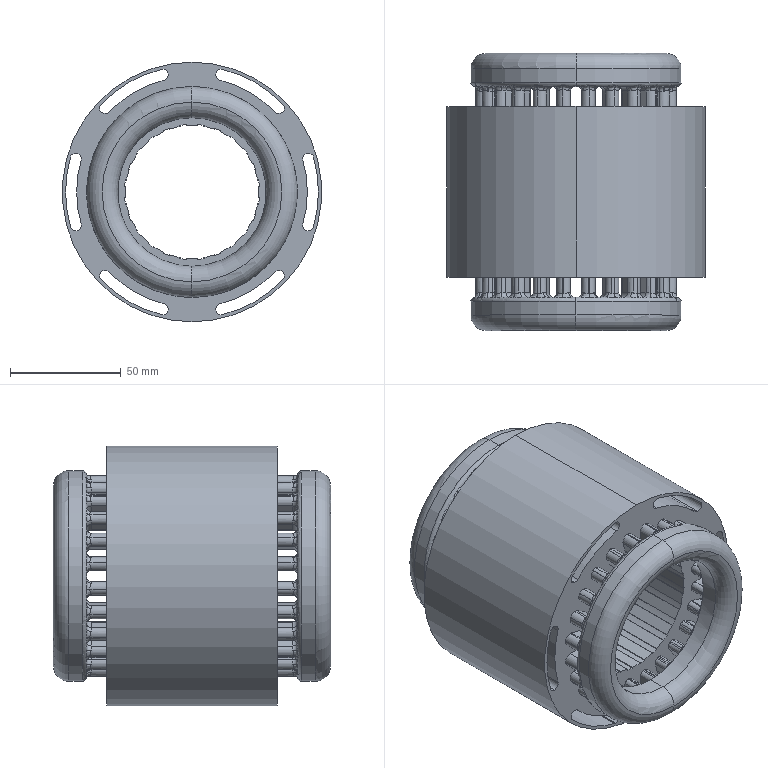Component | SolidWorks | Int_rieur Stator-1 | 1 solid | 1134 faces | box 117 x 125 x 117 mm | volume 646107 mm3 | cylinder 492 | torus 328 | plane 218 | spline 96 | commonest cylinder face diameters 4 x212 6 x120 71 x48 91 x48 61 x24 5 x18 104 x6 114 x6